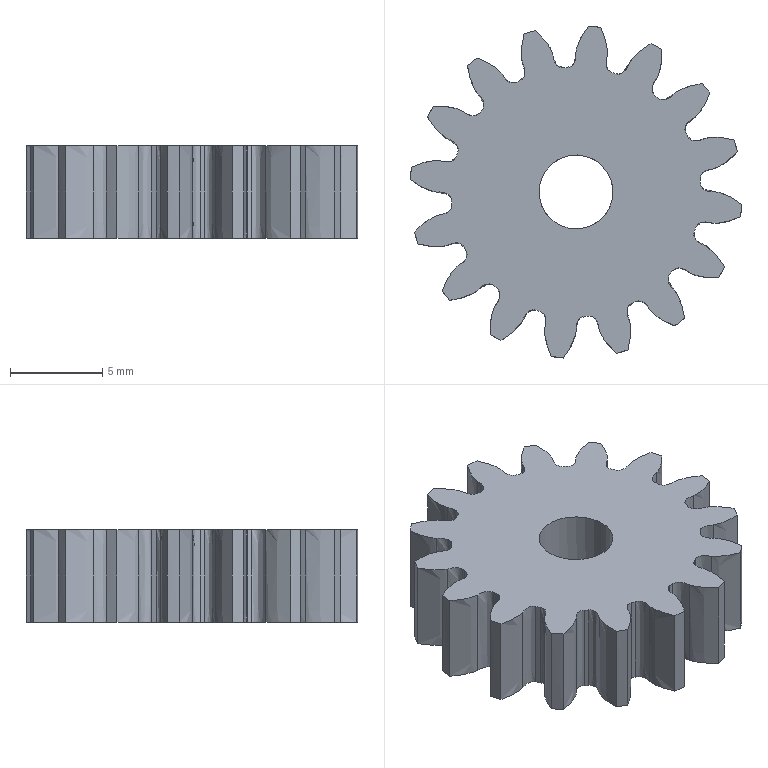Component | NX | GEAR_4 | 1 solid | 99 faces | volume 919 mm3 | other 80 | cylinder 17 | plane 2 | commonest cylinder face diameters 13.5 x16 4 x1